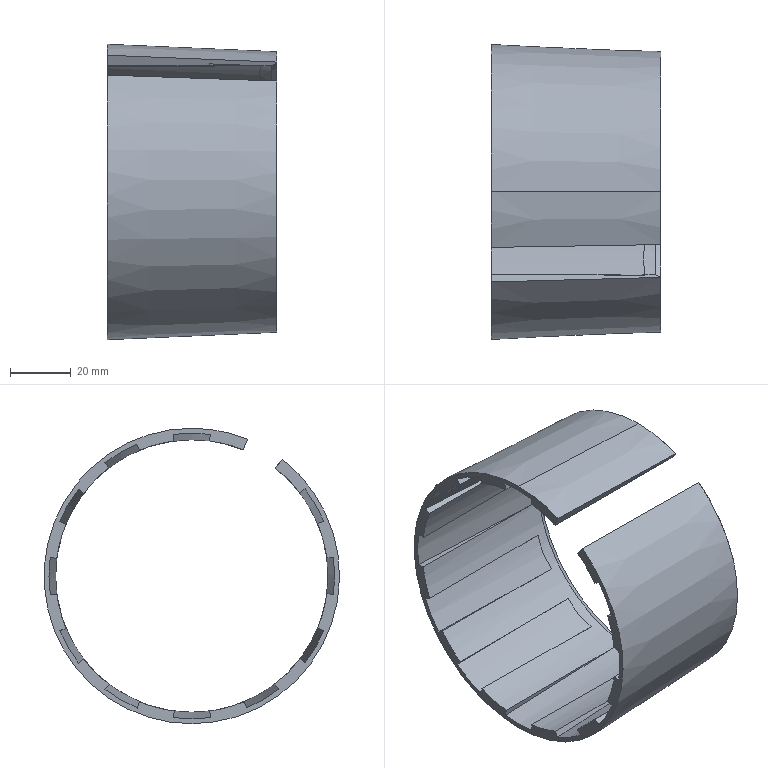Component | SolidWorks | SnapRing-1 | 1 solid | 50 faces | volume 32080 mm3 | plane 28 | spline 13 | cone 6 | cylinder 3 | commonest cylinder face diameters 89.483 x3 | material Plain Carbon Steel